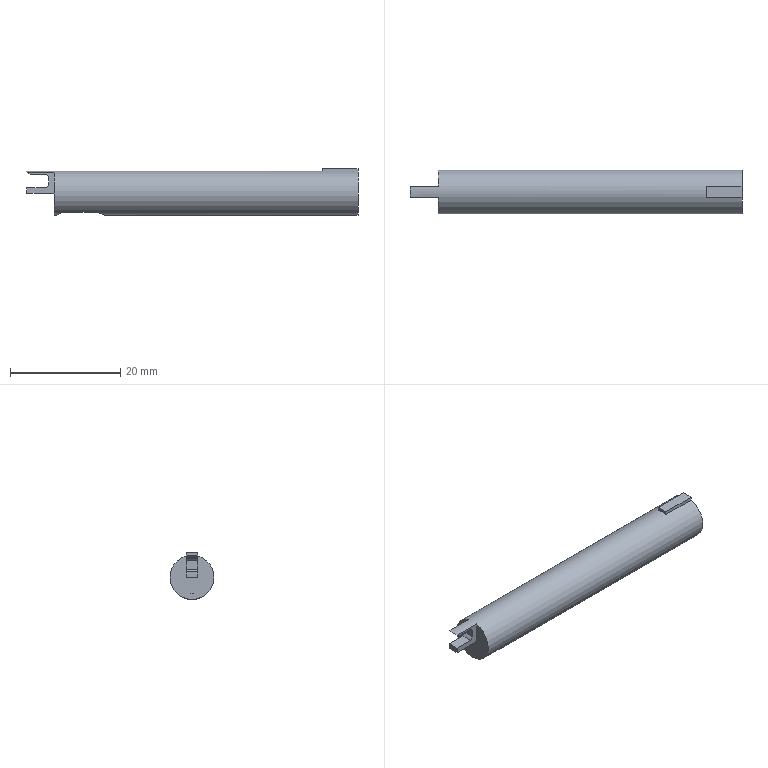Component | NX | SHE_JI-7 | 1 solid | 22 faces | volume 2764 mm3 | plane 19 | cylinder 3 | commonest cylinder face diameters 4 x2 8 x1